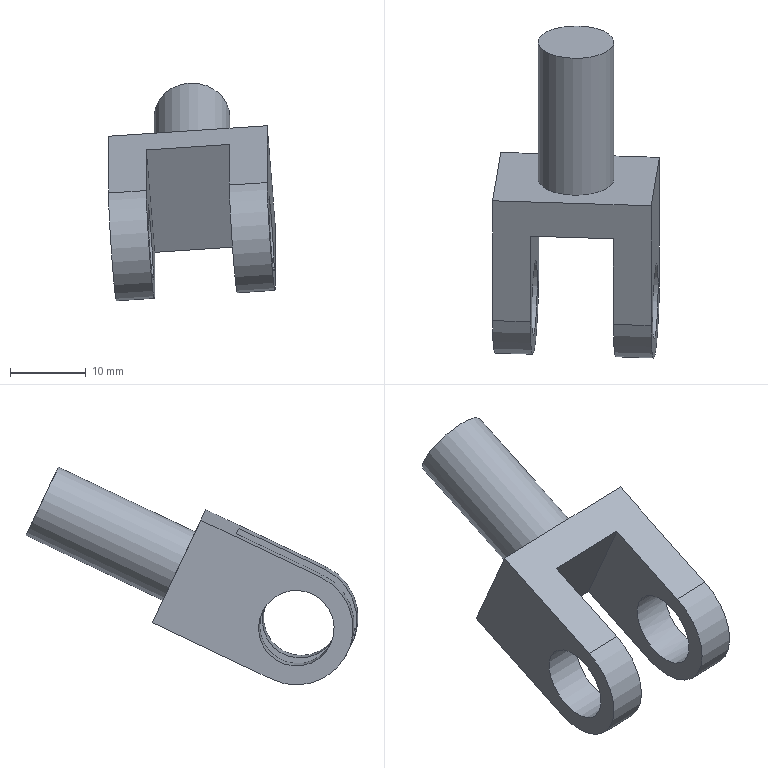Component | NX | JOINT | 1 solid | 14 faces | box 22.04 x 43.85 x 28.77 mm | volume 5119 mm3 | plane 9 | cylinder 5 | commonest cylinder face diameters 10 x3 15 x2
STEP:
#1=CARTESIAN_POINT('',(0.,0.,0.));
#2=DIRECTION('',(0.,0.,1.));
#3=DIRECTION('',(1.,0.,0.));
#4=AXIS2_PLACEMENT_3D('',#1,#2,#3);
#5=CARTESIAN_POINT('',(271.221,-324.741,280.115));
#6=VERTEX_POINT('',#5);
#7=CARTESIAN_POINT('',(271.221,-320.224,282.258));
#8=DIRECTION('',(0.9973,-0.03139,0.06617));
#9=DIRECTION('',(0.,-0.9035,-0.4286));
#10=AXIS2_PLACEMENT_3D('',#7,#8,#9);
#11=CIRCLE('',#10,5.);
#12=CARTESIAN_POINT('',(271.77,-323.794,272.286));
#13=DIRECTION('',(0.9973,-0.03139,0.06617));
#14=DIRECTION('',(-0.07324,-0.4274,0.9011));
#15=AXIS2_PLACEMENT_3D('',#12,#13,#14);
#16=PLANE('',#15);
#17=CARTESIAN_POINT('',(7.5,-7.5));
#18=DIRECTION('',(0.,1.));
#19=AXIS2_PLACEMENT_2D('',#17,#18);
#20=CIRCLE('',#19,5.);
#21=(GEOMETRIC_REPRESENTATION_CONTEXT(2)PARAMETRIC_REPRESENTATION_CONTEXT()REPRESENTATION_CONTEXT('',''));
#22=DEFINITIONAL_REPRESENTATION('',(#20),#21);
#23=PCURVE('',#16,#22);
#24=CARTESIAN_POINT('',(271.221,-320.224,282.258));
#25=DIRECTION('',(0.9973,-0.03139,0.06617));
#26=DIRECTION('',(0.,-0.9035,-0.4286));
#27=AXIS2_PLACEMENT_3D('',#24,#25,#26);
#28=CYLINDRICAL_SURFACE('',#27,5.);
#29=CARTESIAN_POINT('',(0.,0.));
#30=DIRECTION('',(1.,0.));
#31=VECTOR('',#30,1.);
#32=LINE('',#29,#31);
#33=(GEOMETRIC_REPRESENTATION_CONTEXT(2)PARAMETRIC_REPRESENTATION_CONTEXT()REPRESENTATION_CONTEXT('',''));
#34=DEFINITIONAL_REPRESENTATION('',(#32),#33);
#35=PCURVE('',#28,#34);
#36=SURFACE_CURVE('',#11,(#23,#35),.PCURVE_S1.);
#37=EDGE_CURVE('',#6,#6,#36,.T.);
#38=ORIENTED_EDGE('',*,*,#37,.T.);
#39=EDGE_LOOP('',(#38));
#40=FACE_BOUND('',#39,.T.);
#41=CARTESIAN_POINT('',(271.77,-317.018,275.5));
#42=VERTEX_POINT('',#41);
#43=CARTESIAN_POINT('',(270.672,-323.429,289.016));
#44=VERTEX_POINT('',#43);
#45=CARTESIAN_POINT('',(271.221,-320.224,282.258));
#46=DIRECTION('',(-0.9973,0.03139,-0.06617));
#47=DIRECTION('',(-0.07324,-0.4274,0.9011));
#48=AXIS2_PLACEMENT_3D('',#45,#46,#47);
#49=CIRCLE('',#48,7.5);
#50=CARTESIAN_POINT('',(15.,-7.5));
#51=CARTESIAN_POINT('',(15.,-20.49));
#52=CARTESIAN_POINT('',(3.75,-13.995));
#53=CARTESIAN_POINT('',(-7.5,-7.5));
#54=CARTESIAN_POINT('',(3.75,-1.005));
#55=CARTESIAN_POINT('',(15.,5.49));
#56=CARTESIAN_POINT('',(15.,-7.5));
#57=(BOUNDED_CURVE()B_SPLINE_CURVE(2,(#50,#51,#52,#53,#54,#55,#56),.UNSPECIFIED.,.T.,.F.)B_SPLINE_CURVE_WITH_KNOTS((1,2,2,2,2,1),(-2.094,0.,2.094,4.189,6.283,8.378),.UNSPECIFIED.)CURVE()GEOMETRIC_REPRESENTATION_ITEM()RATIONAL_B_SPLINE_CURVE((1.,0.5,1.,0.5,1.,0.5,1.))REPRESENTATION_ITEM(''));
#58=(GEOMETRIC_REPRESENTATION_CONTEXT(2)PARAMETRIC_REPRESENTATION_CONTEXT()REPRESENTATION_CONTEXT('',''));
#59=DEFINITIONAL_REPRESENTATION('',(#57),#58);
#60=PCURVE('',#16,#59);
#61=CARTESIAN_POINT('',(281.693,-320.553,282.953));
#62=DIRECTION('',(0.9973,-0.03139,0.06617));
#63=DIRECTION('',(-0.07324,-0.4274,0.9011));
#64=AXIS2_PLACEMENT_3D('',#61,#62,#63);
#65=CYLINDRICAL_SURFACE('',#64,7.5);
#66=CARTESIAN_POINT('',(6.283,-10.5));
#67=DIRECTION('',(-1.,0.));
#68=VECTOR('',#67,1.);
#69=LINE('',#66,#68);
#70=(GEOMETRIC_REPRESENTATION_CONTEXT(2)PARAMETRIC_REPRESENTATION_CONTEXT()REPRESENTATION_CONTEXT('',''));
#71=DEFINITIONAL_REPRESENTATION('',(#69),#70);
#72=PCURVE('',#65,#71);
#73=SURFACE_CURVE('',#49,(#60,#72),.PCURVE_S1.);
#74=EDGE_CURVE('',#42,#44,#73,.T.);
#75=ORIENTED_EDGE('',*,*,#74,.T.);
#76=CARTESIAN_POINT('',(270.672,-307.618,296.516));
#77=VERTEX_POINT('',#76);
#78=CARTESIAN_POINT('',(270.672,-330.206,285.802));
#79=DIRECTION('',(0.,0.9035,0.4286));
#80=VECTOR('',#79,1.);
#81=LINE('',#78,#80);
#82=CARTESIAN_POINT('',(15.,-0.));
#83=DIRECTION('',(-0.,-1.));
#84=VECTOR('',#83,1.);
#85=LINE('',#82,#84);
#86=(GEOMETRIC_REPRESENTATION_CONTEXT(2)PARAMETRIC_REPRESENTATION_CONTEXT()REPRESENTATION_CONTEXT('',''));
#87=DEFINITIONAL_REPRESENTATION('',(#85),#86);
#88=PCURVE('',#16,#87);
#89=CARTESIAN_POINT('',(281.143,-307.948,297.211));
#90=DIRECTION('',(0.07324,0.4274,-0.9011));
#91=DIRECTION('',(0.9973,-0.03139,0.06617));
#92=AXIS2_PLACEMENT_3D('',#89,#90,#91);
#93=PLANE('',#92);
#94=CARTESIAN_POINT('',(-10.5,25.));
#95=DIRECTION('',(-0.,-1.));
#96=VECTOR('',#95,1.);
#97=LINE('',#94,#96);
#98=(GEOMETRIC_REPRESENTATION_CONTEXT(2)PARAMETRIC_REPRESENTATION_CONTEXT()REPRESENTATION_CONTEXT('',''));
#99=DEFINITIONAL_REPRESENTATION('',(#97),#98);
#100=PCURVE('',#93,#99);
#101=SURFACE_CURVE('',#81,(#88,#100),.PCURVE_S1.);
#102=EDGE_CURVE('',#44,#77,#101,.T.);
#103=ORIENTED_EDGE('',*,*,#102,.T.);
#104=CARTESIAN_POINT('',(271.77,-301.207,283.));
#105=VERTEX_POINT('',#104);
#106=CARTESIAN_POINT('',(271.77,-301.207,283.));
#107=DIRECTION('',(-0.07324,-0.4274,0.9011));
#108=VECTOR('',#107,1.);
#109=LINE('',#106,#108);
#110=CARTESIAN_POINT('',(-0.,-25.));
#111=DIRECTION('',(1.,0.));
#112=VECTOR('',#111,1.);
#113=LINE('',#110,#112);
#114=(GEOMETRIC_REPRESENTATION_CONTEXT(2)PARAMETRIC_REPRESENTATION_CONTEXT()REPRESENTATION_CONTEXT('',''));
#115=DEFINITIONAL_REPRESENTATION('',(#113),#114);
#116=PCURVE('',#16,#115);
#117=CARTESIAN_POINT('',(282.242,-301.536,283.695));
#118=DIRECTION('',(-0.,-0.9035,-0.4286));
#119=DIRECTION('',(-0.9973,0.03139,-0.06617));
#120=AXIS2_PLACEMENT_3D('',#117,#118,#119);
#121=PLANE('',#120);
#122=CARTESIAN_POINT('',(10.5,0.));
#123=DIRECTION('',(0.,-1.));
#124=VECTOR('',#123,1.);
#125=LINE('',#122,#124);
#126=(GEOMETRIC_REPRESENTATION_CONTEXT(2)PARAMETRIC_REPRESENTATION_CONTEXT()REPRESENTATION_CONTEXT('',''));
#127=DEFINITIONAL_REPRESENTATION('',(#125),#126);
#128=PCURVE('',#121,#127);
#129=SURFACE_CURVE('',#109,(#116,#128),.PCURVE_S1.);
#130=EDGE_CURVE('',#105,#77,#129,.T.);
#131=ORIENTED_EDGE('',*,*,#130,.F.);
#132=CARTESIAN_POINT('',(271.77,-323.794,272.286));
#133=DIRECTION('',(0.,0.9035,0.4286));
#134=VECTOR('',#133,1.);
#135=LINE('',#132,#134);
#136=CARTESIAN_POINT('',(0.,0.));
#137=DIRECTION('',(-0.,-1.));
#138=VECTOR('',#137,1.);
#139=LINE('',#136,#138);
#140=(GEOMETRIC_REPRESENTATION_CONTEXT(2)PARAMETRIC_REPRESENTATION_CONTEXT()REPRESENTATION_CONTEXT('',''));
#141=DEFINITIONAL_REPRESENTATION('',(#139),#140);
#142=PCURVE('',#16,#141);
#143=CARTESIAN_POINT('',(282.242,-301.536,283.695));
#144=DIRECTION('',(0.07324,0.4274,-0.9011));
#145=DIRECTION('',(0.9973,-0.03139,0.06617));
#146=AXIS2_PLACEMENT_3D('',#143,#144,#145);
#147=PLANE('',#146);
#148=CARTESIAN_POINT('',(-10.5,25.));
#149=DIRECTION('',(-0.,-1.));
#150=VECTOR('',#149,1.);
#151=LINE('',#148,#150);
#152=(GEOMETRIC_REPRESENTATION_CONTEXT(2)PARAMETRIC_REPRESENTATION_CONTEXT()REPRESENTATION_CONTEXT('',''));
#153=DEFINITIONAL_REPRESENTATION('',(#151),#152);
#154=PCURVE('',#147,#153);
#155=SURFACE_CURVE('',#135,(#142,#154),.PCURVE_S1.);
#156=EDGE_CURVE('',#42,#105,#155,.T.);
#157=ORIENTED_EDGE('',*,*,#156,.F.);
#158=EDGE_LOOP('',(#75,#103,#131,#157));
#159=FACE_BOUND('',#158,.T.);
#160=ADVANCED_FACE('',(#40,#159),#16,.F.);
#161=CARTESIAN_POINT('',(281.327,-306.879,294.958));
#162=VERTEX_POINT('',#161);
#163=CARTESIAN_POINT('',(281.693,-304.742,290.453));
#164=DIRECTION('',(0.,0.9035,0.4286));
#165=DIRECTION('',(-0.07324,-0.4274,0.9011));
#166=AXIS2_PLACEMENT_3D('',#163,#164,#165);
#167=CIRCLE('',#166,5.);
#168=CARTESIAN_POINT('',(-0.,-12.5));
#169=CARTESIAN_POINT('',(-8.66,-12.5));
#170=CARTESIAN_POINT('',(-4.33,-5.));
#171=CARTESIAN_POINT('',(-0.,2.5));
#172=CARTESIAN_POINT('',(4.33,-5.));
#173=CARTESIAN_POINT('',(8.66,-12.5));
#174=CARTESIAN_POINT('',(-0.,-12.5));
#175=(BOUNDED_CURVE()B_SPLINE_CURVE(2,(#168,#169,#170,#171,#172,#173,#174),.UNSPECIFIED.,.T.,.F.)B_SPLINE_CURVE_WITH_KNOTS((1,2,2,2,2,1),(-2.094,0.,2.094,4.189,6.283,8.378),.UNSPECIFIED.)CURVE()GEOMETRIC_REPRESENTATION_ITEM()RATIONAL_B_SPLINE_CURVE((1.,0.5,1.,0.5,1.,0.5,1.))REPRESENTATION_ITEM(''));
#176=(GEOMETRIC_REPRESENTATION_CONTEXT(2)PARAMETRIC_REPRESENTATION_CONTEXT()REPRESENTATION_CONTEXT('',''));
#177=DEFINITIONAL_REPRESENTATION('',(#175),#176);
#178=PCURVE('',#121,#177);
#179=CARTESIAN_POINT('',(281.693,-286.672,299.025));
#180=DIRECTION('',(-0.,-0.9035,-0.4286));
#181=DIRECTION('',(-0.9973,0.03139,-0.06617));
#182=AXIS2_PLACEMENT_3D('',#179,#180,#181);
#183=CYLINDRICAL_SURFACE('',#182,5.);
#184=CARTESIAN_POINT('',(10.996,20.));
#185=DIRECTION('',(-1.,0.));
#186=VECTOR('',#185,1.);
#187=LINE('',#184,#186);
#188=(GEOMETRIC_REPRESENTATION_CONTEXT(2)PARAMETRIC_REPRESENTATION_CONTEXT()REPRESENTATION_CONTEXT('',''));
#189=DEFINITIONAL_REPRESENTATION('',(#187),#188);
#190=PCURVE('',#183,#189);
#191=SURFACE_CURVE('',#167,(#178,#190),.PCURVE_S1.);
#192=EDGE_CURVE('',#162,#162,#191,.T.);
#193=ORIENTED_EDGE('',*,*,#192,.F.);
#194=EDGE_LOOP('',(#193));
#195=FACE_BOUND('',#194,.T.);
#196=CARTESIAN_POINT('',(291.615,-308.277,297.906));
#197=VERTEX_POINT('',#196);
#198=CARTESIAN_POINT('',(281.143,-307.948,297.211));
#199=DIRECTION('',(0.9973,-0.03139,0.06617));
#200=VECTOR('',#199,1.);
#201=LINE('',#198,#200);
#202=CARTESIAN_POINT('',(-0.,-15.));
#203=DIRECTION('',(-1.,0.));
#204=VECTOR('',#203,1.);
#205=LINE('',#202,#204);
#206=(GEOMETRIC_REPRESENTATION_CONTEXT(2)PARAMETRIC_REPRESENTATION_CONTEXT()REPRESENTATION_CONTEXT('',''));
#207=DEFINITIONAL_REPRESENTATION('',(#205),#206);
#208=PCURVE('',#121,#207);
#209=CARTESIAN_POINT('',(0.,0.));
#210=DIRECTION('',(1.,0.));
#211=VECTOR('',#210,1.);
#212=LINE('',#209,#211);
#213=(GEOMETRIC_REPRESENTATION_CONTEXT(2)PARAMETRIC_REPRESENTATION_CONTEXT()REPRESENTATION_CONTEXT('',''));
#214=DEFINITIONAL_REPRESENTATION('',(#212),#213);
#215=PCURVE('',#93,#214);
#216=SURFACE_CURVE('',#201,(#208,#215),.PCURVE_S1.);
#217=EDGE_CURVE('',#77,#197,#216,.T.);
#218=ORIENTED_EDGE('',*,*,#217,.T.);
#219=CARTESIAN_POINT('',(292.714,-301.866,284.39));
#220=VERTEX_POINT('',#219);
#221=CARTESIAN_POINT('',(292.714,-301.866,284.39));
#222=DIRECTION('',(-0.07324,-0.4274,0.9011));
#223=VECTOR('',#222,1.);
#224=LINE('',#221,#223);
#225=CARTESIAN_POINT('',(-10.5,0.));
#226=DIRECTION('',(0.,-1.));
#227=VECTOR('',#226,1.);
#228=LINE('',#225,#227);
#229=(GEOMETRIC_REPRESENTATION_CONTEXT(2)PARAMETRIC_REPRESENTATION_CONTEXT()REPRESENTATION_CONTEXT('',''));
#230=DEFINITIONAL_REPRESENTATION('',(#228),#229);
#231=PCURVE('',#121,#230);
#232=CARTESIAN_POINT('',(292.714,-301.866,284.39));
#233=DIRECTION('',(-0.9973,0.03139,-0.06617));
#234=DIRECTION('',(0.07324,0.4274,-0.9011));
#235=AXIS2_PLACEMENT_3D('',#232,#233,#234);
#236=PLANE('',#235);
#237=CARTESIAN_POINT('',(0.,0.));
#238=DIRECTION('',(-1.,0.));
#239=VECTOR('',#238,1.);
#240=LINE('',#237,#239);
#241=(GEOMETRIC_REPRESENTATION_CONTEXT(2)PARAMETRIC_REPRESENTATION_CONTEXT()REPRESENTATION_CONTEXT('',''));
#242=DEFINITIONAL_REPRESENTATION('',(#240),#241);
#243=PCURVE('',#236,#242);
#244=SURFACE_CURVE('',#224,(#231,#243),.PCURVE_S1.);
#245=EDGE_CURVE('',#220,#197,#244,.T.);
#246=ORIENTED_EDGE('',*,*,#245,.F.);
#247=CARTESIAN_POINT('',(271.77,-301.207,283.));
#248=DIRECTION('',(0.9973,-0.03139,0.06617));
#249=VECTOR('',#248,1.);
#250=LINE('',#247,#249);
#251=CARTESIAN_POINT('',(10.5,0.));
#252=DIRECTION('',(-1.,-0.));
#253=VECTOR('',#252,1.);
#254=LINE('',#251,#253);
#255=(GEOMETRIC_REPRESENTATION_CONTEXT(2)PARAMETRIC_REPRESENTATION_CONTEXT()REPRESENTATION_CONTEXT('',''));
#256=DEFINITIONAL_REPRESENTATION('',(#254),#255);
#257=PCURVE('',#121,#256);
#258=CARTESIAN_POINT('',(-10.5,0.));
#259=DIRECTION('',(1.,-0.));
#260=VECTOR('',#259,1.);
#261=LINE('',#258,#260);
#262=(GEOMETRIC_REPRESENTATION_CONTEXT(2)PARAMETRIC_REPRESENTATION_CONTEXT()REPRESENTATION_CONTEXT('',''));
#263=DEFINITIONAL_REPRESENTATION('',(#261),#262);
#264=PCURVE('',#147,#263);
#265=SURFACE_CURVE('',#250,(#257,#264),.PCURVE_S1.);
#266=EDGE_CURVE('',#105,#220,#265,.T.);
#267=ORIENTED_EDGE('',*,*,#266,.F.);
#268=ORIENTED_EDGE('',*,*,#130,.T.);
#269=EDGE_LOOP('',(#218,#246,#267,#268));
#270=FACE_BOUND('',#269,.T.);
#271=ADVANCED_FACE('',(#195,#270),#121,.F.);
#272=CARTESIAN_POINT('',(292.531,-318.746,279.142));
#273=VERTEX_POINT('',#272);
#274=CARTESIAN_POINT('',(292.165,-325.4,281.505));
#275=VERTEX_POINT('',#274);
#276=CARTESIAN_POINT('',(292.165,-320.883,283.648));
#277=DIRECTION('',(-0.9973,0.03139,-0.06617));
#278=DIRECTION('',(0.07324,0.4274,-0.9011));
#279=AXIS2_PLACEMENT_3D('',#276,#277,#278);
#280=CIRCLE('',#279,5.);
#281=CARTESIAN_POINT('',(-7.5,17.5));
#282=DIRECTION('',(1.,-0.));
#283=AXIS2_PLACEMENT_2D('',#281,#282);
#284=CIRCLE('',#283,5.);
#285=(GEOMETRIC_REPRESENTATION_CONTEXT(2)PARAMETRIC_REPRESENTATION_CONTEXT()REPRESENTATION_CONTEXT('',''));
#286=DEFINITIONAL_REPRESENTATION('',(#284),#285);
#287=PCURVE('',#236,#286);
#288=CARTESIAN_POINT('',(271.221,-320.224,282.258));
#289=DIRECTION('',(0.9973,-0.03139,0.06617));
#290=DIRECTION('',(0.,-0.9035,-0.4286));
#291=AXIS2_PLACEMENT_3D('',#288,#289,#290);
#292=CYLINDRICAL_SURFACE('',#291,5.);
#293=CARTESIAN_POINT('',(1.571,21.));
#294=DIRECTION('',(-1.,0.));
#295=VECTOR('',#294,1.);
#296=LINE('',#293,#295);
#297=(GEOMETRIC_REPRESENTATION_CONTEXT(2)PARAMETRIC_REPRESENTATION_CONTEXT()REPRESENTATION_CONTEXT('',''));
#298=DEFINITIONAL_REPRESENTATION('',(#296),#297);
#299=PCURVE('',#292,#298);
#300=SURFACE_CURVE('',#280,(#287,#299),.PCURVE_S1.);
#301=EDGE_CURVE('',#273,#275,#300,.T.);
#302=ORIENTED_EDGE('',*,*,#301,.T.);
#303=CARTESIAN_POINT('',(292.165,-320.883,283.648));
#304=DIRECTION('',(-0.9973,0.03139,-0.06617));
#305=DIRECTION('',(0.07324,0.4274,-0.9011));
#306=AXIS2_PLACEMENT_3D('',#303,#304,#305);
#307=CIRCLE('',#306,5.);
#308=CARTESIAN_POINT('',(-7.5,17.5));
#309=DIRECTION('',(1.,-0.));
#310=AXIS2_PLACEMENT_2D('',#308,#309);
#311=CIRCLE('',#310,5.);
#312=(GEOMETRIC_REPRESENTATION_CONTEXT(2)PARAMETRIC_REPRESENTATION_CONTEXT()REPRESENTATION_CONTEXT('',''));
#313=DEFINITIONAL_REPRESENTATION('',(#311),#312);
#314=PCURVE('',#236,#313);
#315=CARTESIAN_POINT('',(7.854,21.));
#316=DIRECTION('',(-1.,0.));
#317=VECTOR('',#316,1.);
#318=LINE('',#315,#317);
#319=(GEOMETRIC_REPRESENTATION_CONTEXT(2)PARAMETRIC_REPRESENTATION_CONTEXT()REPRESENTATION_CONTEXT('',''));
#320=DEFINITIONAL_REPRESENTATION('',(#318),#319);
#321=PCURVE('',#292,#320);
#322=SURFACE_CURVE('',#307,(#314,#321),.PCURVE_S1.);
#323=EDGE_CURVE('',#275,#273,#322,.T.);
#324=ORIENTED_EDGE('',*,*,#323,.T.);
#325=EDGE_LOOP('',(#302,#324));
#326=FACE_BOUND('',#325,.T.);
#327=CARTESIAN_POINT('',(291.615,-324.089,290.406));
#328=VERTEX_POINT('',#327);
#329=CARTESIAN_POINT('',(291.615,-308.277,297.906));
#330=DIRECTION('',(0.,-0.9035,-0.4286));
#331=VECTOR('',#330,1.);
#332=LINE('',#329,#331);
#333=CARTESIAN_POINT('',(-15.,-0.));
#334=DIRECTION('',(-0.,1.));
#335=VECTOR('',#334,1.);
#336=LINE('',#333,#335);
#337=(GEOMETRIC_REPRESENTATION_CONTEXT(2)PARAMETRIC_REPRESENTATION_CONTEXT()REPRESENTATION_CONTEXT('',''));
#338=DEFINITIONAL_REPRESENTATION('',(#336),#337);
#339=PCURVE('',#236,#338);
#340=CARTESIAN_POINT('',(10.5,-0.));
#341=DIRECTION('',(0.,1.));
#342=VECTOR('',#341,1.);
#343=LINE('',#340,#342);
#344=(GEOMETRIC_REPRESENTATION_CONTEXT(2)PARAMETRIC_REPRESENTATION_CONTEXT()REPRESENTATION_CONTEXT('',''));
#345=DEFINITIONAL_REPRESENTATION('',(#343),#344);
#346=PCURVE('',#93,#345);
#347=SURFACE_CURVE('',#332,(#339,#346),.PCURVE_S1.);
#348=EDGE_CURVE('',#197,#328,#347,.T.);
#349=ORIENTED_EDGE('',*,*,#348,.T.);
#350=CARTESIAN_POINT('',(292.714,-317.677,276.89));
#351=VERTEX_POINT('',#350);
#352=CARTESIAN_POINT('',(292.165,-320.883,283.648));
#353=DIRECTION('',(0.9973,-0.03139,0.06617));
#354=DIRECTION('',(0.07324,0.4274,-0.9011));
#355=AXIS2_PLACEMENT_3D('',#352,#353,#354);
#356=CIRCLE('',#355,7.5);
#357=CARTESIAN_POINT('',(0.,17.5));
#358=CARTESIAN_POINT('',(0.,4.51));
#359=CARTESIAN_POINT('',(-11.25,11.005));
#360=CARTESIAN_POINT('',(-22.5,17.5));
#361=CARTESIAN_POINT('',(-11.25,23.995));
#362=CARTESIAN_POINT('',(0.,30.49));
#363=CARTESIAN_POINT('',(0.,17.5));
#364=(BOUNDED_CURVE()B_SPLINE_CURVE(2,(#357,#358,#359,#360,#361,#362,#363),.UNSPECIFIED.,.T.,.F.)B_SPLINE_CURVE_WITH_KNOTS((1,2,2,2,2,1),(-2.094,0.,2.094,4.189,6.283,8.378),.UNSPECIFIED.)CURVE()GEOMETRIC_REPRESENTATION_ITEM()RATIONAL_B_SPLINE_CURVE((1.,0.5,1.,0.5,1.,0.5,1.))REPRESENTATION_ITEM(''));
#365=(GEOMETRIC_REPRESENTATION_CONTEXT(2)PARAMETRIC_REPRESENTATION_CONTEXT()REPRESENTATION_CONTEXT('',''));
#366=DEFINITIONAL_REPRESENTATION('',(#364),#365);
#367=PCURVE('',#236,#366);
#368=CARTESIAN_POINT('',(281.693,-320.553,282.953));
#369=DIRECTION('',(0.9973,-0.03139,0.06617));
#370=DIRECTION('',(-0.07324,-0.4274,0.9011));
#371=AXIS2_PLACEMENT_3D('',#368,#369,#370);
#372=CYLINDRICAL_SURFACE('',#371,7.5);
#373=CARTESIAN_POINT('',(-3.142,10.5));
#374=DIRECTION('',(1.,0.));
#375=VECTOR('',#374,1.);
#376=LINE('',#373,#375);
#377=(GEOMETRIC_REPRESENTATION_CONTEXT(2)PARAMETRIC_REPRESENTATION_CONTEXT()REPRESENTATION_CONTEXT('',''));
#378=DEFINITIONAL_REPRESENTATION('',(#376),#377);
#379=PCURVE('',#372,#378);
#380=SURFACE_CURVE('',#356,(#367,#379),.PCURVE_S1.);
#381=EDGE_CURVE('',#328,#351,#380,.T.);
#382=ORIENTED_EDGE('',*,*,#381,.T.);
#383=CARTESIAN_POINT('',(292.714,-301.866,284.39));
#384=DIRECTION('',(0.,-0.9035,-0.4286));
#385=VECTOR('',#384,1.);
#386=LINE('',#383,#385);
#387=CARTESIAN_POINT('',(0.,0.));
#388=DIRECTION('',(-0.,1.));
#389=VECTOR('',#388,1.);
#390=LINE('',#387,#389);
#391=(GEOMETRIC_REPRESENTATION_CONTEXT(2)PARAMETRIC_REPRESENTATION_CONTEXT()REPRESENTATION_CONTEXT('',''));
#392=DEFINITIONAL_REPRESENTATION('',(#390),#391);
#393=PCURVE('',#236,#392);
#394=CARTESIAN_POINT('',(10.5,0.));
#395=DIRECTION('',(0.,1.));
#396=VECTOR('',#395,1.);
#397=LINE('',#394,#396);
#398=(GEOMETRIC_REPRESENTATION_CONTEXT(2)PARAMETRIC_REPRESENTATION_CONTEXT()REPRESENTATION_CONTEXT('',''));
#399=DEFINITIONAL_REPRESENTATION('',(#397),#398);
#400=PCURVE('',#147,#399);
#401=SURFACE_CURVE('',#386,(#393,#400),.PCURVE_S1.);
#402=EDGE_CURVE('',#220,#351,#401,.T.);
#403=ORIENTED_EDGE('',*,*,#402,.F.);
#404=ORIENTED_EDGE('',*,*,#245,.T.);
#405=EDGE_LOOP('',(#349,#382,#403,#404));
#406=FACE_BOUND('',#405,.T.);
#407=ADVANCED_FACE('',(#326,#406),#236,.F.);
#408=CARTESIAN_POINT('',(287.178,-325.243,281.174));
#409=VERTEX_POINT('',#408);
#410=CARTESIAN_POINT('',(287.178,-320.726,283.317));
#411=DIRECTION('',(0.9973,-0.03139,0.06617));
#412=DIRECTION('',(0.,-0.9035,-0.4286));
#413=AXIS2_PLACEMENT_3D('',#410,#411,#412);
#414=CIRCLE('',#413,5.);
#415=CARTESIAN_POINT('',(287.727,-324.296,273.344));
#416=DIRECTION('',(0.9973,-0.03139,0.06617));
#417=DIRECTION('',(0.,-0.9035,-0.4286));
#418=AXIS2_PLACEMENT_3D('',#415,#416,#417);
#419=PLANE('',#418);
#420=CARTESIAN_POINT('',(-7.5,-7.5));
#421=DIRECTION('',(1.,-0.));
#422=AXIS2_PLACEMENT_2D('',#420,#421);
#423=CIRCLE('',#422,5.);
#424=(GEOMETRIC_REPRESENTATION_CONTEXT(2)PARAMETRIC_REPRESENTATION_CONTEXT()REPRESENTATION_CONTEXT('',''));
#425=DEFINITIONAL_REPRESENTATION('',(#423),#424);
#426=PCURVE('',#419,#425);
#427=CARTESIAN_POINT('',(0.,16.));
#428=DIRECTION('',(1.,0.));
#429=VECTOR('',#428,1.);
#430=LINE('',#427,#429);
#431=(GEOMETRIC_REPRESENTATION_CONTEXT(2)PARAMETRIC_REPRESENTATION_CONTEXT()REPRESENTATION_CONTEXT('',''));
#432=DEFINITIONAL_REPRESENTATION('',(#430),#431);
#433=PCURVE('',#292,#432);
#434=SURFACE_CURVE('',#414,(#426,#433),.PCURVE_S1.);
#435=EDGE_CURVE('',#409,#409,#434,.T.);
#436=ORIENTED_EDGE('',*,*,#435,.T.);
#437=EDGE_LOOP('',(#436));
#438=FACE_BOUND('',#437,.T.);
#439=CARTESIAN_POINT('',(287.727,-317.52,276.559));
#440=VERTEX_POINT('',#439);
#441=CARTESIAN_POINT('',(286.629,-323.932,290.075));
#442=VERTEX_POINT('',#441);
#443=CARTESIAN_POINT('',(287.178,-320.726,283.317));
#444=DIRECTION('',(-0.9973,0.03139,-0.06617));
#445=DIRECTION('',(0.,-0.9035,-0.4286));
#446=AXIS2_PLACEMENT_3D('',#443,#444,#445);
#447=CIRCLE('',#446,7.5);
#448=CARTESIAN_POINT('',(-0.,-7.5));
#449=CARTESIAN_POINT('',(-0.,-20.49));
#450=CARTESIAN_POINT('',(-11.25,-13.995));
#451=CARTESIAN_POINT('',(-22.5,-7.5));
#452=CARTESIAN_POINT('',(-11.25,-1.005));
#453=CARTESIAN_POINT('',(-0.,5.49));
#454=CARTESIAN_POINT('',(-0.,-7.5));
#455=(BOUNDED_CURVE()B_SPLINE_CURVE(2,(#448,#449,#450,#451,#452,#453,#454),.UNSPECIFIED.,.T.,.F.)B_SPLINE_CURVE_WITH_KNOTS((1,2,2,2,2,1),(-2.094,0.,2.094,4.189,6.283,8.378),.UNSPECIFIED.)CURVE()GEOMETRIC_REPRESENTATION_ITEM()RATIONAL_B_SPLINE_CURVE((1.,0.5,1.,0.5,1.,0.5,1.))REPRESENTATION_ITEM(''));
#456=(GEOMETRIC_REPRESENTATION_CONTEXT(2)PARAMETRIC_REPRESENTATION_CONTEXT()REPRESENTATION_CONTEXT('',''));
#457=DEFINITIONAL_REPRESENTATION('',(#455),#456);
#458=PCURVE('',#419,#457);
#459=CARTESIAN_POINT('',(7.854,5.5));
#460=DIRECTION('',(-1.,0.));
#461=VECTOR('',#460,1.);
#462=LINE('',#459,#461);
#463=(GEOMETRIC_REPRESENTATION_CONTEXT(2)PARAMETRIC_REPRESENTATION_CONTEXT()REPRESENTATION_CONTEXT('',''));
#464=DEFINITIONAL_REPRESENTATION('',(#462),#463);
#465=PCURVE('',#372,#464);
#466=SURFACE_CURVE('',#447,(#458,#465),.PCURVE_S1.);
#467=EDGE_CURVE('',#440,#442,#466,.T.);
#468=ORIENTED_EDGE('',*,*,#467,.T.);
#469=CARTESIAN_POINT('',(286.629,-312.638,295.432));
#470=VERTEX_POINT('',#469);
#471=CARTESIAN_POINT('',(286.629,-330.708,286.86));
#472=DIRECTION('',(-0.,0.9035,0.4286));
#473=VECTOR('',#472,1.);
#474=LINE('',#471,#473);
#475=CARTESIAN_POINT('',(-0.,-15.));
#476=DIRECTION('',(-1.,0.));
#477=VECTOR('',#476,1.);
#478=LINE('',#475,#477);
#479=(GEOMETRIC_REPRESENTATION_CONTEXT(2)PARAMETRIC_REPRESENTATION_CONTEXT()REPRESENTATION_CONTEXT('',''));
#480=DEFINITIONAL_REPRESENTATION('',(#478),#479);
#481=PCURVE('',#419,#480);
#482=CARTESIAN_POINT('',(5.5,25.));
#483=DIRECTION('',(-0.,-1.));
#484=VECTOR('',#483,1.);
#485=LINE('',#482,#484);
#486=(GEOMETRIC_REPRESENTATION_CONTEXT(2)PARAMETRIC_REPRESENTATION_CONTEXT()REPRESENTATION_CONTEXT('',''));
#487=DEFINITIONAL_REPRESENTATION('',(#485),#486);
#488=PCURVE('',#93,#487);
#489=SURFACE_CURVE('',#474,(#481,#488),.PCURVE_S1.);
#490=EDGE_CURVE('',#442,#470,#489,.T.);
#491=ORIENTED_EDGE('',*,*,#490,.T.);
#492=CARTESIAN_POINT('',(287.727,-306.226,281.916));
#493=VERTEX_POINT('',#492);
#494=CARTESIAN_POINT('',(287.727,-306.226,281.916));
#495=DIRECTION('',(-0.07324,-0.4274,0.9011));
#496=VECTOR('',#495,1.);
#497=LINE('',#494,#496);
#498=CARTESIAN_POINT('',(-20.,-0.));
#499=DIRECTION('',(0.,-1.));
#500=VECTOR('',#499,1.);
#501=LINE('',#498,#500);
#502=(GEOMETRIC_REPRESENTATION_CONTEXT(2)PARAMETRIC_REPRESENTATION_CONTEXT()REPRESENTATION_CONTEXT('',''));
#503=DEFINITIONAL_REPRESENTATION('',(#501),#502);
#504=PCURVE('',#419,#503);
#505=CARTESIAN_POINT('',(282.242,-306.054,281.552));
#506=DIRECTION('',(0.,0.9035,0.4286));
#507=DIRECTION('',(-0.07324,-0.4274,0.9011));
#508=AXIS2_PLACEMENT_3D('',#505,#506,#507);
#509=PLANE('',#508);
#510=CARTESIAN_POINT('',(-0.,5.5));
#511=DIRECTION('',(1.,0.));
#512=VECTOR('',#511,1.);
#513=LINE('',#510,#512);
#514=(GEOMETRIC_REPRESENTATION_CONTEXT(2)PARAMETRIC_REPRESENTATION_CONTEXT()REPRESENTATION_CONTEXT('',''));
#515=DEFINITIONAL_REPRESENTATION('',(#513),#514);
#516=PCURVE('',#509,#515);
#517=SURFACE_CURVE('',#497,(#504,#516),.PCURVE_S1.);
#518=EDGE_CURVE('',#493,#470,#517,.T.);
#519=ORIENTED_EDGE('',*,*,#518,.F.);
#520=CARTESIAN_POINT('',(287.727,-324.296,273.344));
#521=DIRECTION('',(-0.,0.9035,0.4286));
#522=VECTOR('',#521,1.);
#523=LINE('',#520,#522);
#524=CARTESIAN_POINT('',(0.,0.));
#525=DIRECTION('',(-1.,0.));
#526=VECTOR('',#525,1.);
#527=LINE('',#524,#526);
#528=(GEOMETRIC_REPRESENTATION_CONTEXT(2)PARAMETRIC_REPRESENTATION_CONTEXT()REPRESENTATION_CONTEXT('',''));
#529=DEFINITIONAL_REPRESENTATION('',(#527),#528);
#530=PCURVE('',#419,#529);
#531=CARTESIAN_POINT('',(5.5,25.));
#532=DIRECTION('',(-0.,-1.));
#533=VECTOR('',#532,1.);
#534=LINE('',#531,#533);
#535=(GEOMETRIC_REPRESENTATION_CONTEXT(2)PARAMETRIC_REPRESENTATION_CONTEXT()REPRESENTATION_CONTEXT('',''));
#536=DEFINITIONAL_REPRESENTATION('',(#534),#535);
#537=PCURVE('',#147,#536);
#538=SURFACE_CURVE('',#523,(#530,#537),.PCURVE_S1.);
#539=EDGE_CURVE('',#440,#493,#538,.T.);
#540=ORIENTED_EDGE('',*,*,#539,.F.);
#541=EDGE_LOOP('',(#468,#491,#519,#540));
#542=FACE_BOUND('',#541,.T.);
#543=ADVANCED_FACE('',(#438,#542),#419,.F.);
#544=CARTESIAN_POINT('',(275.658,-312.293,294.704));
#545=VERTEX_POINT('',#544);
#546=CARTESIAN_POINT('',(281.143,-312.465,295.068));
#547=DIRECTION('',(-0.9973,0.03139,-0.06617));
#548=VECTOR('',#547,1.);
#549=LINE('',#546,#548);
#550=CARTESIAN_POINT('',(15.,0.));
#551=DIRECTION('',(0.,-1.));
#552=VECTOR('',#551,1.);
#553=LINE('',#550,#552);
#554=(GEOMETRIC_REPRESENTATION_CONTEXT(2)PARAMETRIC_REPRESENTATION_CONTEXT()REPRESENTATION_CONTEXT('',''));
#555=DEFINITIONAL_REPRESENTATION('',(#553),#554);
#556=PCURVE('',#509,#555);
#557=CARTESIAN_POINT('',(0.,5.));
#558=DIRECTION('',(-1.,0.));
#559=VECTOR('',#558,1.);
#560=LINE('',#557,#559);
#561=(GEOMETRIC_REPRESENTATION_CONTEXT(2)PARAMETRIC_REPRESENTATION_CONTEXT()REPRESENTATION_CONTEXT('',''));
#562=DEFINITIONAL_REPRESENTATION('',(#560),#561);
#563=PCURVE('',#93,#562);
#564=SURFACE_CURVE('',#549,(#556,#563),.PCURVE_S1.);
#565=EDGE_CURVE('',#470,#545,#564,.T.);
#566=ORIENTED_EDGE('',*,*,#565,.T.);
#567=CARTESIAN_POINT('',(276.757,-305.881,281.188));
#568=VERTEX_POINT('',#567);
#569=CARTESIAN_POINT('',(276.757,-305.881,281.188));
#570=DIRECTION('',(-0.07324,-0.4274,0.9011));
#571=VECTOR('',#570,1.);
#572=LINE('',#569,#571);
#573=CARTESIAN_POINT('',(0.,-5.5));
#574=DIRECTION('',(1.,0.));
#575=VECTOR('',#574,1.);
#576=LINE('',#573,#575);
#577=(GEOMETRIC_REPRESENTATION_CONTEXT(2)PARAMETRIC_REPRESENTATION_CONTEXT()REPRESENTATION_CONTEXT('',''));
#578=DEFINITIONAL_REPRESENTATION('',(#576),#577);
#579=PCURVE('',#509,#578);
#580=CARTESIAN_POINT('',(276.757,-305.881,281.188));
#581=DIRECTION('',(-0.9973,0.03139,-0.06617));
#582=DIRECTION('',(0.,0.9035,0.4286));
#583=AXIS2_PLACEMENT_3D('',#580,#581,#582);
#584=PLANE('',#583);
#585=CARTESIAN_POINT('',(0.,0.));
#586=DIRECTION('',(-0.,-1.));
#587=VECTOR('',#586,1.);
#588=LINE('',#585,#587);
#589=(GEOMETRIC_REPRESENTATION_CONTEXT(2)PARAMETRIC_REPRESENTATION_CONTEXT()REPRESENTATION_CONTEXT('',''));
#590=DEFINITIONAL_REPRESENTATION('',(#588),#589);
#591=PCURVE('',#584,#590);
#592=SURFACE_CURVE('',#572,(#579,#591),.PCURVE_S1.);
#593=EDGE_CURVE('',#568,#545,#592,.T.);
#594=ORIENTED_EDGE('',*,*,#593,.F.);
#595=CARTESIAN_POINT('',(287.727,-306.226,281.916));
#596=DIRECTION('',(-0.9973,0.03139,-0.06617));
#597=VECTOR('',#596,1.);
#598=LINE('',#595,#597);
#599=CARTESIAN_POINT('',(-0.,5.5));
#600=DIRECTION('',(0.,-1.));
#601=VECTOR('',#600,1.);
#602=LINE('',#599,#601);
#603=(GEOMETRIC_REPRESENTATION_CONTEXT(2)PARAMETRIC_REPRESENTATION_CONTEXT()REPRESENTATION_CONTEXT('',''));
#604=DEFINITIONAL_REPRESENTATION('',(#602),#603);
#605=PCURVE('',#509,#604);
#606=CARTESIAN_POINT('',(5.5,5.));
#607=DIRECTION('',(-1.,0.));
#608=VECTOR('',#607,1.);
#609=LINE('',#606,#608);
#610=(GEOMETRIC_REPRESENTATION_CONTEXT(2)PARAMETRIC_REPRESENTATION_CONTEXT()REPRESENTATION_CONTEXT('',''));
#611=DEFINITIONAL_REPRESENTATION('',(#609),#610);
#612=PCURVE('',#147,#611);
#613=SURFACE_CURVE('',#598,(#605,#612),.PCURVE_S1.);
#614=EDGE_CURVE('',#493,#568,#613,.T.);
#615=ORIENTED_EDGE('',*,*,#614,.F.);
#616=ORIENTED_EDGE('',*,*,#518,.T.);
#617=EDGE_LOOP('',(#566,#594,#615,#616));
#618=FACE_BOUND('',#617,.T.);
#619=ADVANCED_FACE('',(#618),#509,.F.);
#620=CARTESIAN_POINT('',(276.208,-315.863,284.732));
#621=VERTEX_POINT('',#620);
#622=CARTESIAN_POINT('',(276.208,-324.898,280.446));
#623=VERTEX_POINT('',#622);
#624=CARTESIAN_POINT('',(276.208,-320.381,282.589));
#625=DIRECTION('',(-0.9973,0.03139,-0.06617));
#626=DIRECTION('',(0.,0.9035,0.4286));
#627=AXIS2_PLACEMENT_3D('',#624,#625,#626);
#628=CIRCLE('',#627,5.);
#629=CARTESIAN_POINT('',(-12.5,-7.5));
#630=DIRECTION('',(1.,0.));
#631=AXIS2_PLACEMENT_2D('',#629,#630);
#632=CIRCLE('',#631,5.);
#633=(GEOMETRIC_REPRESENTATION_CONTEXT(2)PARAMETRIC_REPRESENTATION_CONTEXT()REPRESENTATION_CONTEXT('',''));
#634=DEFINITIONAL_REPRESENTATION('',(#632),#633);
#635=PCURVE('',#584,#634);
#636=CARTESIAN_POINT('',(3.142,5.));
#637=DIRECTION('',(-1.,0.));
#638=VECTOR('',#637,1.);
#639=LINE('',#636,#638);
#640=(GEOMETRIC_REPRESENTATION_CONTEXT(2)PARAMETRIC_REPRESENTATION_CONTEXT()REPRESENTATION_CONTEXT('',''));
#641=DEFINITIONAL_REPRESENTATION('',(#639),#640);
#642=PCURVE('',#28,#641);
#643=SURFACE_CURVE('',#628,(#635,#642),.PCURVE_S1.);
#644=EDGE_CURVE('',#621,#623,#643,.T.);
#645=ORIENTED_EDGE('',*,*,#644,.T.);
#646=CARTESIAN_POINT('',(276.208,-320.381,282.589));
#647=DIRECTION('',(-0.9973,0.03139,-0.06617));
#648=DIRECTION('',(0.,0.9035,0.4286));
#649=AXIS2_PLACEMENT_3D('',#646,#647,#648);
#650=CIRCLE('',#649,5.);
#651=CARTESIAN_POINT('',(-12.5,-7.5));
#652=DIRECTION('',(1.,0.));
#653=AXIS2_PLACEMENT_2D('',#651,#652);
#654=CIRCLE('',#653,5.);
#655=(GEOMETRIC_REPRESENTATION_CONTEXT(2)PARAMETRIC_REPRESENTATION_CONTEXT()REPRESENTATION_CONTEXT('',''));
#656=DEFINITIONAL_REPRESENTATION('',(#654),#655);
#657=PCURVE('',#584,#656);
#658=CARTESIAN_POINT('',(9.425,5.));
#659=DIRECTION('',(-1.,0.));
#660=VECTOR('',#659,1.);
#661=LINE('',#658,#660);
#662=(GEOMETRIC_REPRESENTATION_CONTEXT(2)PARAMETRIC_REPRESENTATION_CONTEXT()REPRESENTATION_CONTEXT('',''));
#663=DEFINITIONAL_REPRESENTATION('',(#661),#662);
#664=PCURVE('',#28,#663);
#665=SURFACE_CURVE('',#650,(#657,#664),.PCURVE_S1.);
#666=EDGE_CURVE('',#623,#621,#665,.T.);
#667=ORIENTED_EDGE('',*,*,#666,.T.);
#668=EDGE_LOOP('',(#645,#667));
#669=FACE_BOUND('',#668,.T.);
#670=CARTESIAN_POINT('',(275.658,-323.586,289.347));
#671=VERTEX_POINT('',#670);
#672=CARTESIAN_POINT('',(275.658,-312.293,294.704));
#673=DIRECTION('',(-0.,-0.9035,-0.4286));
#674=VECTOR('',#673,1.);
#675=LINE('',#672,#674);
#676=CARTESIAN_POINT('',(0.,-15.));
#677=DIRECTION('',(-1.,-0.));
#678=VECTOR('',#677,1.);
#679=LINE('',#676,#678);
#680=(GEOMETRIC_REPRESENTATION_CONTEXT(2)PARAMETRIC_REPRESENTATION_CONTEXT()REPRESENTATION_CONTEXT('',''));
#681=DEFINITIONAL_REPRESENTATION('',(#679),#680);
#682=PCURVE('',#584,#681);
#683=CARTESIAN_POINT('',(-5.5,5.));
#684=DIRECTION('',(-0.,1.));
#685=VECTOR('',#684,1.);
#686=LINE('',#683,#685);
#687=(GEOMETRIC_REPRESENTATION_CONTEXT(2)PARAMETRIC_REPRESENTATION_CONTEXT()REPRESENTATION_CONTEXT('',''));
#688=DEFINITIONAL_REPRESENTATION('',(#686),#687);
#689=PCURVE('',#93,#688);
#690=SURFACE_CURVE('',#675,(#682,#689),.PCURVE_S1.);
#691=EDGE_CURVE('',#545,#671,#690,.T.);
#692=ORIENTED_EDGE('',*,*,#691,.T.);
#693=CARTESIAN_POINT('',(276.757,-317.175,275.831));
#694=VERTEX_POINT('',#693);
#695=CARTESIAN_POINT('',(276.208,-320.381,282.589));
#696=DIRECTION('',(0.9973,-0.03139,0.06617));
#697=DIRECTION('',(0.,0.9035,0.4286));
#698=AXIS2_PLACEMENT_3D('',#695,#696,#697);
#699=CIRCLE('',#698,7.5);
#700=CARTESIAN_POINT('',(-5.,-7.5));
#701=CARTESIAN_POINT('',(-5.,-20.49));
#702=CARTESIAN_POINT('',(-16.25,-13.995));
#703=CARTESIAN_POINT('',(-27.5,-7.5));
#704=CARTESIAN_POINT('',(-16.25,-1.005));
#705=CARTESIAN_POINT('',(-5.,5.49));
#706=CARTESIAN_POINT('',(-5.,-7.5));
#707=(BOUNDED_CURVE()B_SPLINE_CURVE(2,(#700,#701,#702,#703,#704,#705,#706),.UNSPECIFIED.,.T.,.F.)B_SPLINE_CURVE_WITH_KNOTS((1,2,2,2,2,1),(-2.094,0.,2.094,4.189,6.283,8.378),.UNSPECIFIED.)CURVE()GEOMETRIC_REPRESENTATION_ITEM()RATIONAL_B_SPLINE_CURVE((1.,0.5,1.,0.5,1.,0.5,1.))REPRESENTATION_ITEM(''));
#708=(GEOMETRIC_REPRESENTATION_CONTEXT(2)PARAMETRIC_REPRESENTATION_CONTEXT()REPRESENTATION_CONTEXT('',''));
#709=DEFINITIONAL_REPRESENTATION('',(#707),#708);
#710=PCURVE('',#584,#709);
#711=CARTESIAN_POINT('',(-1.571,-5.5));
#712=DIRECTION('',(1.,0.));
#713=VECTOR('',#712,1.);
#714=LINE('',#711,#713);
#715=(GEOMETRIC_REPRESENTATION_CONTEXT(2)PARAMETRIC_REPRESENTATION_CONTEXT()REPRESENTATION_CONTEXT('',''));
#716=DEFINITIONAL_REPRESENTATION('',(#714),#715);
#717=PCURVE('',#65,#716);
#718=SURFACE_CURVE('',#699,(#710,#717),.PCURVE_S1.);
#719=EDGE_CURVE('',#671,#694,#718,.T.);
#720=ORIENTED_EDGE('',*,*,#719,.T.);
#721=CARTESIAN_POINT('',(276.757,-305.881,281.188));
#722=DIRECTION('',(-0.,-0.9035,-0.4286));
#723=VECTOR('',#722,1.);
#724=LINE('',#721,#723);
#725=CARTESIAN_POINT('',(0.,0.));
#726=DIRECTION('',(-1.,-0.));
#727=VECTOR('',#726,1.);
#728=LINE('',#725,#727);
#729=(GEOMETRIC_REPRESENTATION_CONTEXT(2)PARAMETRIC_REPRESENTATION_CONTEXT()REPRESENTATION_CONTEXT('',''));
#730=DEFINITIONAL_REPRESENTATION('',(#728),#729);
#731=PCURVE('',#584,#730);
#732=CARTESIAN_POINT('',(-5.5,5.));
#733=DIRECTION('',(-0.,1.));
#734=VECTOR('',#733,1.);
#735=LINE('',#732,#734);
#736=(GEOMETRIC_REPRESENTATION_CONTEXT(2)PARAMETRIC_REPRESENTATION_CONTEXT()REPRESENTATION_CONTEXT('',''));
#737=DEFINITIONAL_REPRESENTATION('',(#735),#736);
#738=PCURVE('',#147,#737);
#739=SURFACE_CURVE('',#724,(#731,#738),.PCURVE_S1.);
#740=EDGE_CURVE('',#568,#694,#739,.T.);
#741=ORIENTED_EDGE('',*,*,#740,.F.);
#742=ORIENTED_EDGE('',*,*,#593,.T.);
#743=EDGE_LOOP('',(#692,#720,#741,#742));
#744=FACE_BOUND('',#743,.T.);
#745=ADVANCED_FACE('',(#669,#744),#584,.F.);
#746=ORIENTED_EDGE('',*,*,#402,.T.);
#747=CARTESIAN_POINT('',(287.727,-317.52,276.559));
#748=DIRECTION('',(-0.9973,0.03139,-0.06617));
#749=VECTOR('',#748,1.);
#750=LINE('',#747,#749);
#751=CARTESIAN_POINT('',(5.5,17.5));
#752=DIRECTION('',(-1.,0.));
#753=VECTOR('',#752,1.);
#754=LINE('',#751,#753);
#755=(GEOMETRIC_REPRESENTATION_CONTEXT(2)PARAMETRIC_REPRESENTATION_CONTEXT()REPRESENTATION_CONTEXT('',''));
#756=DEFINITIONAL_REPRESENTATION('',(#754),#755);
#757=PCURVE('',#147,#756);
#758=CARTESIAN_POINT('',(3.142,5.5));
#759=DIRECTION('',(-0.,-1.));
#760=VECTOR('',#759,1.);
#761=LINE('',#758,#760);
#762=(GEOMETRIC_REPRESENTATION_CONTEXT(2)PARAMETRIC_REPRESENTATION_CONTEXT()REPRESENTATION_CONTEXT('',''));
#763=DEFINITIONAL_REPRESENTATION('',(#761),#762);
#764=PCURVE('',#372,#763);
#765=SURFACE_CURVE('',#750,(#757,#764),.PCURVE_S1.);
#766=EDGE_CURVE('',#351,#440,#765,.T.);
#767=ORIENTED_EDGE('',*,*,#766,.T.);
#768=ORIENTED_EDGE('',*,*,#539,.T.);
#769=ORIENTED_EDGE('',*,*,#614,.T.);
#770=ORIENTED_EDGE('',*,*,#740,.T.);
#771=CARTESIAN_POINT('',(271.77,-317.018,275.5));
#772=DIRECTION('',(-0.9973,0.03139,-0.06617));
#773=VECTOR('',#772,1.);
#774=LINE('',#771,#773);
#775=CARTESIAN_POINT('',(-10.5,17.5));
#776=DIRECTION('',(-1.,0.));
#777=VECTOR('',#776,1.);
#778=LINE('',#775,#777);
#779=(GEOMETRIC_REPRESENTATION_CONTEXT(2)PARAMETRIC_REPRESENTATION_CONTEXT()REPRESENTATION_CONTEXT('',''));
#780=DEFINITIONAL_REPRESENTATION('',(#778),#779);
#781=PCURVE('',#147,#780);
#782=CARTESIAN_POINT('',(3.142,-10.5));
#783=DIRECTION('',(-0.,-1.));
#784=VECTOR('',#783,1.);
#785=LINE('',#782,#784);
#786=(GEOMETRIC_REPRESENTATION_CONTEXT(2)PARAMETRIC_REPRESENTATION_CONTEXT()REPRESENTATION_CONTEXT('',''));
#787=DEFINITIONAL_REPRESENTATION('',(#785),#786);
#788=PCURVE('',#65,#787);
#789=SURFACE_CURVE('',#774,(#781,#788),.PCURVE_S1.);
#790=EDGE_CURVE('',#694,#42,#789,.T.);
#791=ORIENTED_EDGE('',*,*,#790,.T.);
#792=ORIENTED_EDGE('',*,*,#156,.T.);
#793=ORIENTED_EDGE('',*,*,#266,.T.);
#794=EDGE_LOOP('',(#746,#767,#768,#769,#770,#791,#792,#793));
#795=FACE_BOUND('',#794,.T.);
#796=ADVANCED_FACE('',(#795),#147,.T.);
#797=ORIENTED_EDGE('',*,*,#490,.F.);
#798=CARTESIAN_POINT('',(281.143,-323.759,289.711));
#799=DIRECTION('',(0.9973,-0.03139,0.06617));
#800=VECTOR('',#799,1.);
#801=LINE('',#798,#800);
#802=CARTESIAN_POINT('',(-0.,17.5));
#803=DIRECTION('',(1.,0.));
#804=VECTOR('',#803,1.);
#805=LINE('',#802,#804);
#806=(GEOMETRIC_REPRESENTATION_CONTEXT(2)PARAMETRIC_REPRESENTATION_CONTEXT()REPRESENTATION_CONTEXT('',''));
#807=DEFINITIONAL_REPRESENTATION('',(#805),#806);
#808=PCURVE('',#93,#807);
#809=CARTESIAN_POINT('',(0.,0.));
#810=DIRECTION('',(0.,1.));
#811=VECTOR('',#810,1.);
#812=LINE('',#809,#811);
#813=(GEOMETRIC_REPRESENTATION_CONTEXT(2)PARAMETRIC_REPRESENTATION_CONTEXT()REPRESENTATION_CONTEXT('',''));
#814=DEFINITIONAL_REPRESENTATION('',(#812),#813);
#815=PCURVE('',#372,#814);
#816=SURFACE_CURVE('',#801,(#808,#815),.PCURVE_S1.);
#817=EDGE_CURVE('',#442,#328,#816,.T.);
#818=ORIENTED_EDGE('',*,*,#817,.T.);
#819=ORIENTED_EDGE('',*,*,#348,.F.);
#820=ORIENTED_EDGE('',*,*,#217,.F.);
#821=ORIENTED_EDGE('',*,*,#102,.F.);
#822=CARTESIAN_POINT('',(281.143,-323.759,289.711));
#823=DIRECTION('',(0.9973,-0.03139,0.06617));
#824=VECTOR('',#823,1.);
#825=LINE('',#822,#824);
#826=CARTESIAN_POINT('',(-0.,17.5));
#827=DIRECTION('',(1.,0.));
#828=VECTOR('',#827,1.);
#829=LINE('',#826,#828);
#830=(GEOMETRIC_REPRESENTATION_CONTEXT(2)PARAMETRIC_REPRESENTATION_CONTEXT()REPRESENTATION_CONTEXT('',''));
#831=DEFINITIONAL_REPRESENTATION('',(#829),#830);
#832=PCURVE('',#93,#831);
#833=CARTESIAN_POINT('',(0.,0.));
#834=DIRECTION('',(0.,1.));
#835=VECTOR('',#834,1.);
#836=LINE('',#833,#835);
#837=(GEOMETRIC_REPRESENTATION_CONTEXT(2)PARAMETRIC_REPRESENTATION_CONTEXT()REPRESENTATION_CONTEXT('',''));
#838=DEFINITIONAL_REPRESENTATION('',(#836),#837);
#839=PCURVE('',#65,#838);
#840=SURFACE_CURVE('',#825,(#832,#839),.PCURVE_S1.);
#841=EDGE_CURVE('',#44,#671,#840,.T.);
#842=ORIENTED_EDGE('',*,*,#841,.T.);
#843=ORIENTED_EDGE('',*,*,#691,.F.);
#844=ORIENTED_EDGE('',*,*,#565,.F.);
#845=EDGE_LOOP('',(#797,#818,#819,#820,#821,#842,#843,#844));
#846=FACE_BOUND('',#845,.T.);
#847=ADVANCED_FACE('',(#846),#93,.F.);
#848=ORIENTED_EDGE('',*,*,#719,.F.);
#849=ORIENTED_EDGE('',*,*,#841,.F.);
#850=ORIENTED_EDGE('',*,*,#74,.F.);
#851=ORIENTED_EDGE('',*,*,#790,.F.);
#852=EDGE_LOOP('',(#848,#849,#850,#851));
#853=FACE_BOUND('',#852,.T.);
#854=ADVANCED_FACE('',(#853),#65,.T.);
#855=ORIENTED_EDGE('',*,*,#766,.F.);
#856=ORIENTED_EDGE('',*,*,#381,.F.);
#857=ORIENTED_EDGE('',*,*,#817,.F.);
#858=ORIENTED_EDGE('',*,*,#467,.F.);
#859=EDGE_LOOP('',(#855,#856,#857,#858));
#860=FACE_BOUND('',#859,.T.);
#861=ADVANCED_FACE('',(#860),#372,.T.);
#862=ORIENTED_EDGE('',*,*,#37,.T.);
#863=CARTESIAN_POINT('',(271.221,-324.741,280.115));
#864=CARTESIAN_POINT('',(276.208,-324.898,280.446));
#865=B_SPLINE_CURVE_WITH_KNOTS('',1,(#863,#864),.UNSPECIFIED.,.F.,.F.,(2,2),(0.,5.),.PIECEWISE_BEZIER_KNOTS.);
#866=CARTESIAN_POINT('',(6.283,0.));
#867=DIRECTION('',(0.,1.));
#868=VECTOR('',#867,1.);
#869=LINE('',#866,#868);
#870=(GEOMETRIC_REPRESENTATION_CONTEXT(2)PARAMETRIC_REPRESENTATION_CONTEXT()REPRESENTATION_CONTEXT('',''));
#871=DEFINITIONAL_REPRESENTATION('',(#869),#870);
#872=PCURVE('',#28,#871);
#873=CARTESIAN_POINT('',(0.,0.));
#874=DIRECTION('',(0.,1.));
#875=VECTOR('',#874,1.);
#876=LINE('',#873,#875);
#877=(GEOMETRIC_REPRESENTATION_CONTEXT(2)PARAMETRIC_REPRESENTATION_CONTEXT()REPRESENTATION_CONTEXT('',''));
#878=DEFINITIONAL_REPRESENTATION('',(#876),#877);
#879=PCURVE('',#28,#878);
#880=SEAM_CURVE('',#865,(#872,#879),.PCURVE_S1.);
#881=EDGE_CURVE('',#6,#623,#880,.T.);
#882=ORIENTED_EDGE('',*,*,#881,.T.);
#883=ORIENTED_EDGE('',*,*,#666,.T.);
#884=ORIENTED_EDGE('',*,*,#644,.T.);
#885=ORIENTED_EDGE('',*,*,#881,.F.);
#886=EDGE_LOOP('',(#862,#882,#883,#884,#885));
#887=FACE_BOUND('',#886,.F.);
#888=ADVANCED_FACE('',(#887),#28,.F.);
#889=ORIENTED_EDGE('',*,*,#435,.T.);
#890=CARTESIAN_POINT('',(287.178,-325.243,281.174));
#891=CARTESIAN_POINT('',(292.165,-325.4,281.505));
#892=B_SPLINE_CURVE_WITH_KNOTS('',1,(#890,#891),.UNSPECIFIED.,.F.,.F.,(2,2),(16.,21.),.PIECEWISE_BEZIER_KNOTS.);
#893=CARTESIAN_POINT('',(6.283,0.));
#894=DIRECTION('',(0.,1.));
#895=VECTOR('',#894,1.);
#896=LINE('',#893,#895);
#897=(GEOMETRIC_REPRESENTATION_CONTEXT(2)PARAMETRIC_REPRESENTATION_CONTEXT()REPRESENTATION_CONTEXT('',''));
#898=DEFINITIONAL_REPRESENTATION('',(#896),#897);
#899=PCURVE('',#292,#898);
#900=CARTESIAN_POINT('',(0.,0.));
#901=DIRECTION('',(0.,1.));
#902=VECTOR('',#901,1.);
#903=LINE('',#900,#902);
#904=(GEOMETRIC_REPRESENTATION_CONTEXT(2)PARAMETRIC_REPRESENTATION_CONTEXT()REPRESENTATION_CONTEXT('',''));
#905=DEFINITIONAL_REPRESENTATION('',(#903),#904);
#906=PCURVE('',#292,#905);
#907=SEAM_CURVE('',#892,(#899,#906),.PCURVE_S1.);
#908=EDGE_CURVE('',#409,#275,#907,.T.);
#909=ORIENTED_EDGE('',*,*,#908,.T.);
#910=ORIENTED_EDGE('',*,*,#323,.T.);
#911=ORIENTED_EDGE('',*,*,#301,.T.);
#912=ORIENTED_EDGE('',*,*,#908,.F.);
#913=EDGE_LOOP('',(#889,#909,#910,#911,#912));
#914=FACE_BOUND('',#913,.F.);
#915=ADVANCED_FACE('',(#914),#292,.F.);
#916=CARTESIAN_POINT('',(281.327,-288.809,303.53));
#917=VERTEX_POINT('',#916);
#918=CARTESIAN_POINT('',(281.693,-286.672,299.025));
#919=DIRECTION('',(0.,0.9035,0.4286));
#920=DIRECTION('',(-0.07324,-0.4274,0.9011));
#921=AXIS2_PLACEMENT_3D('',#918,#919,#920);
#922=CIRCLE('',#921,5.);
#923=CARTESIAN_POINT('',(10.996,0.));
#924=DIRECTION('',(-1.,0.));
#925=VECTOR('',#924,1.);
#926=LINE('',#923,#925);
#927=(GEOMETRIC_REPRESENTATION_CONTEXT(2)PARAMETRIC_REPRESENTATION_CONTEXT()REPRESENTATION_CONTEXT('',''));
#928=DEFINITIONAL_REPRESENTATION('',(#926),#927);
#929=PCURVE('',#183,#928);
#930=CARTESIAN_POINT('',(281.693,-286.672,299.025));
#931=DIRECTION('',(0.,0.9035,0.4286));
#932=DIRECTION('',(0.9973,-0.03139,0.06617));
#933=AXIS2_PLACEMENT_3D('',#930,#931,#932);
#934=PLANE('',#933);
#935=CARTESIAN_POINT('',(0.,0.));
#936=DIRECTION('',(0.,-1.));
#937=AXIS2_PLACEMENT_2D('',#935,#936);
#938=CIRCLE('',#937,5.);
#939=(GEOMETRIC_REPRESENTATION_CONTEXT(2)PARAMETRIC_REPRESENTATION_CONTEXT()REPRESENTATION_CONTEXT('',''));
#940=DEFINITIONAL_REPRESENTATION('',(#938),#939);
#941=PCURVE('',#934,#940);
#942=SURFACE_CURVE('',#922,(#929,#941),.PCURVE_S1.);
#943=EDGE_CURVE('',#917,#917,#942,.T.);
#944=ORIENTED_EDGE('',*,*,#943,.F.);
#945=CARTESIAN_POINT('',(281.327,-288.809,303.53));
#946=CARTESIAN_POINT('',(281.327,-306.879,294.958));
#947=B_SPLINE_CURVE_WITH_KNOTS('',1,(#945,#946),.UNSPECIFIED.,.F.,.F.,(2,2),(0.,20.),.PIECEWISE_BEZIER_KNOTS.);
#948=CARTESIAN_POINT('',(10.996,0.));
#949=DIRECTION('',(0.,1.));
#950=VECTOR('',#949,1.);
#951=LINE('',#948,#950);
#952=(GEOMETRIC_REPRESENTATION_CONTEXT(2)PARAMETRIC_REPRESENTATION_CONTEXT()REPRESENTATION_CONTEXT('',''));
#953=DEFINITIONAL_REPRESENTATION('',(#951),#952);
#954=PCURVE('',#183,#953);
#955=CARTESIAN_POINT('',(4.712,0.));
#956=DIRECTION('',(0.,1.));
#957=VECTOR('',#956,1.);
#958=LINE('',#955,#957);
#959=(GEOMETRIC_REPRESENTATION_CONTEXT(2)PARAMETRIC_REPRESENTATION_CONTEXT()REPRESENTATION_CONTEXT('',''));
#960=DEFINITIONAL_REPRESENTATION('',(#958),#959);
#961=PCURVE('',#183,#960);
#962=SEAM_CURVE('',#947,(#954,#961),.PCURVE_S1.);
#963=EDGE_CURVE('',#917,#162,#962,.T.);
#964=ORIENTED_EDGE('',*,*,#963,.T.);
#965=ORIENTED_EDGE('',*,*,#192,.T.);
#966=ORIENTED_EDGE('',*,*,#963,.F.);
#967=EDGE_LOOP('',(#944,#964,#965,#966));
#968=FACE_BOUND('',#967,.T.);
#969=ADVANCED_FACE('',(#968),#183,.T.);
#970=ORIENTED_EDGE('',*,*,#943,.T.);
#971=EDGE_LOOP('',(#970));
#972=FACE_BOUND('',#971,.T.);
#973=ADVANCED_FACE('',(#972),#934,.T.);
#974=CLOSED_SHELL('',(#160,#271,#407,#543,#619,#745,#796,#847,#854,#861,#888,#915,#969,#973));
#975=MANIFOLD_SOLID_BREP('',#974);
#976=(LENGTH_UNIT()NAMED_UNIT(*)SI_UNIT(.MILLI.,.METRE.));
#977=UNCERTAINTY_MEASURE_WITH_UNIT(LENGTH_MEASURE(0.000002),#976,'','');
#978=(NAMED_UNIT(*)PLANE_ANGLE_UNIT()SI_UNIT($,.RADIAN.));
#979=(NAMED_UNIT(*)SI_UNIT($,.STERADIAN.)SOLID_ANGLE_UNIT());
#980=(GEOMETRIC_REPRESENTATION_CONTEXT(3)GLOBAL_UNCERTAINTY_ASSIGNED_CONTEXT((#977))GLOBAL_UNIT_ASSIGNED_CONTEXT((#976,#978,#979))REPRESENTATION_CONTEXT('',''));
#981=ADVANCED_BREP_SHAPE_REPRESENTATION('',(#4,#975),#980);